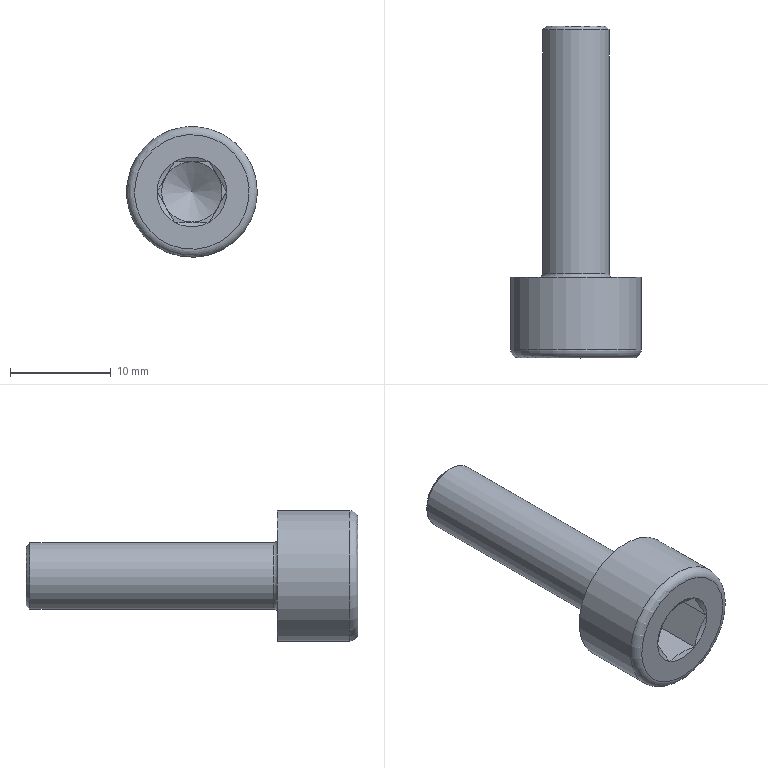Component | NX | SCREW_M8X25 | 1 solid | 27 faces | volume 1752 mm3 | plane 15 | cone 8 | cylinder 2 | torus 2 | commonest cylinder face diameters 6.619 x1 13 x1